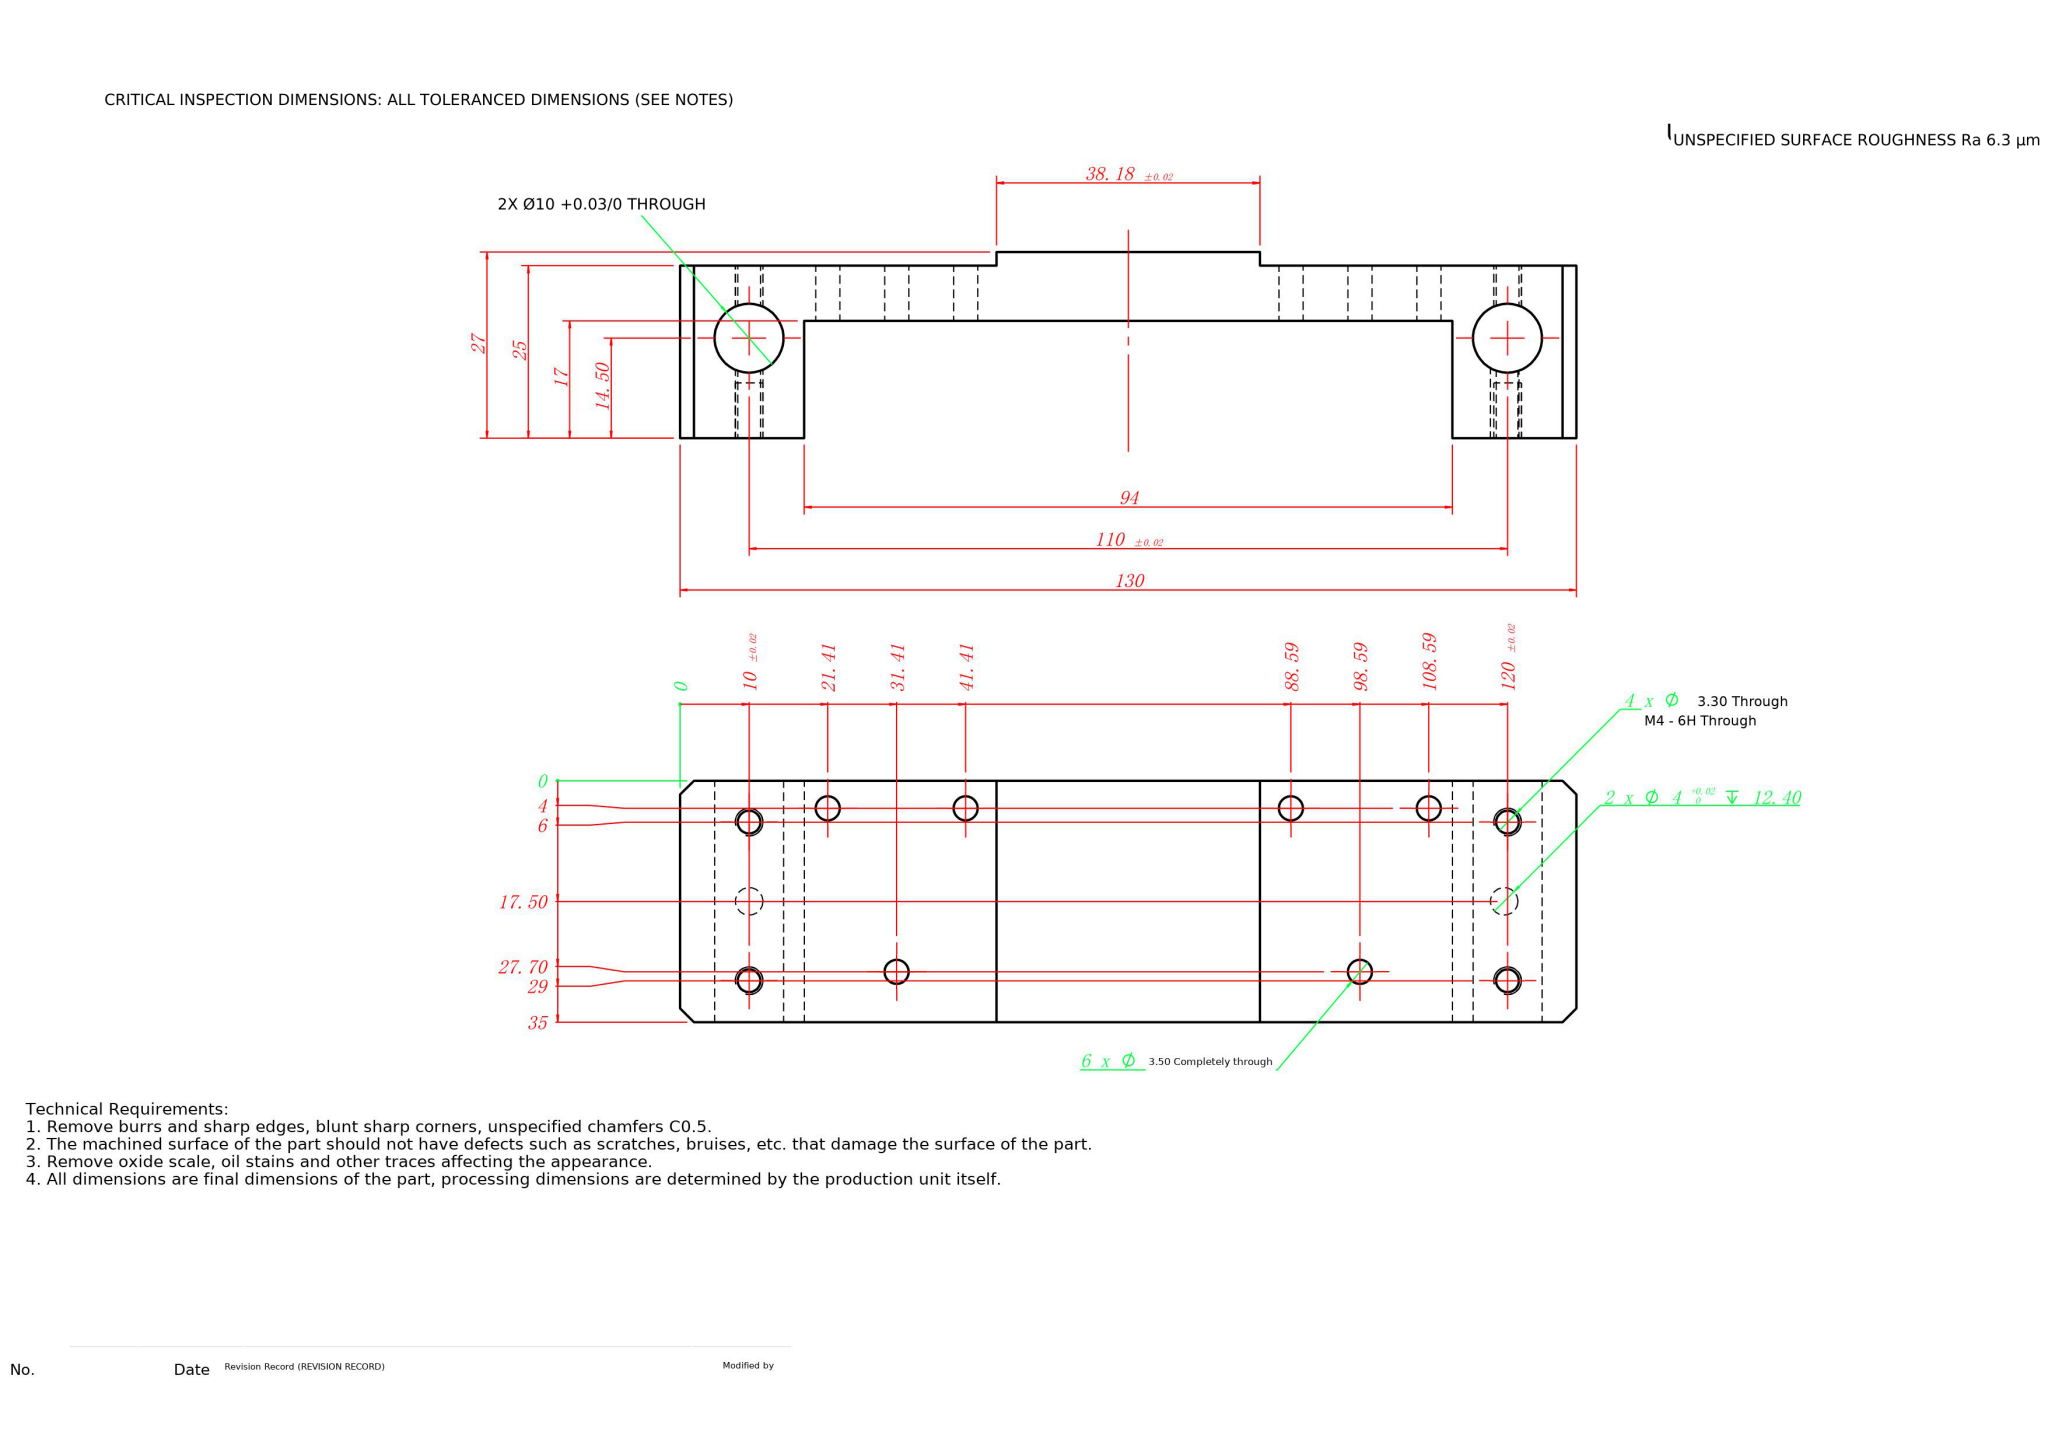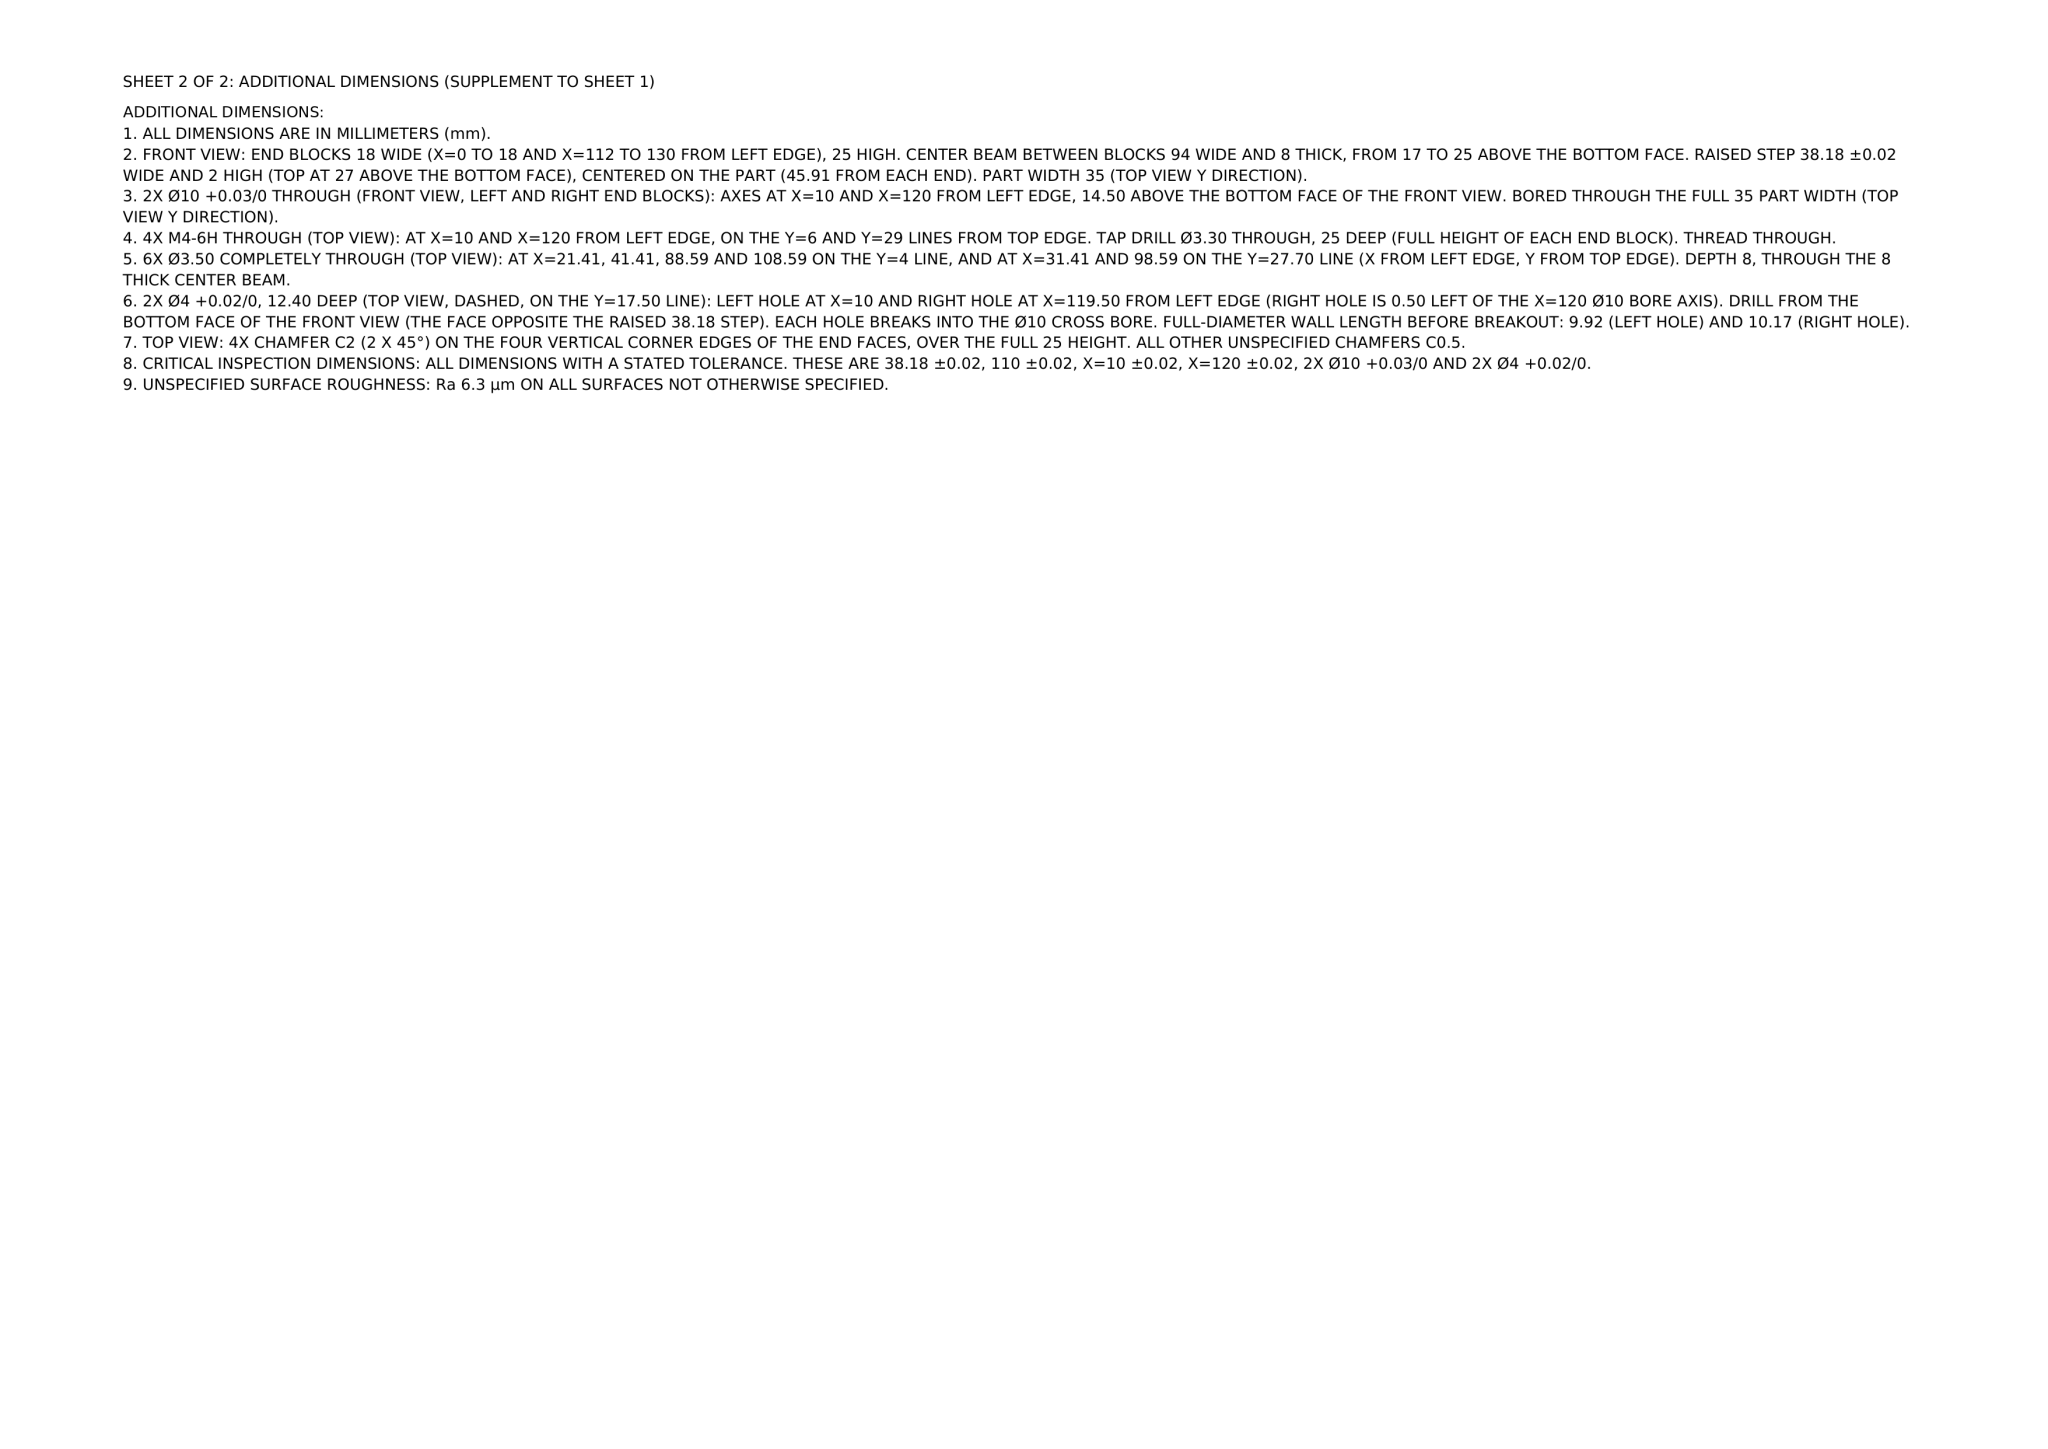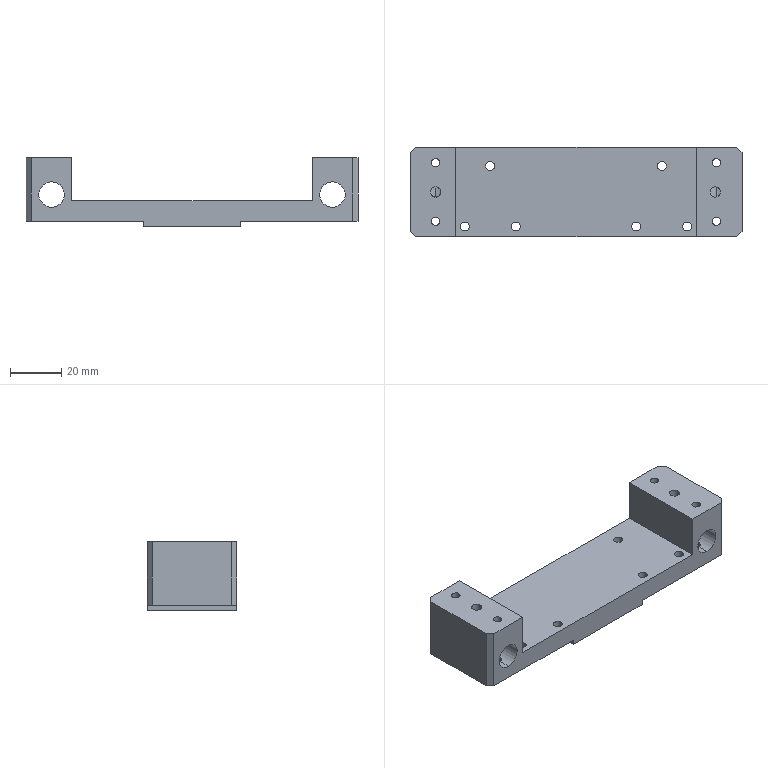Part | NX | mm | 1 solid | 54 faces | box 130 x 35 x 27 mm | volume 53573 mm3 | cylinder 36 | plane 18 | commonest cylinder face diameters 3.3 x16 3.5 x12 4 x4 10 x4